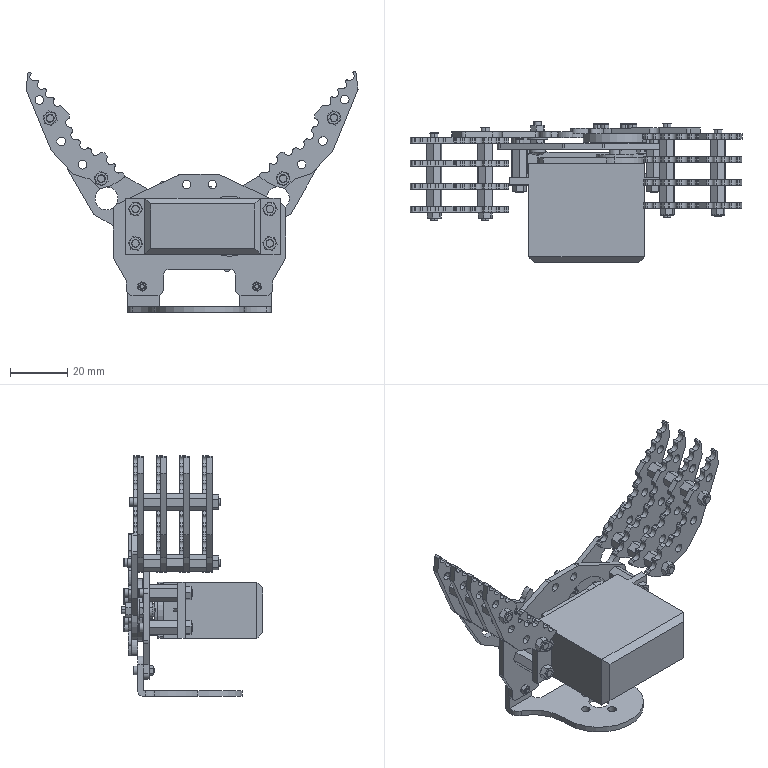Assembly | SolidWorks | mm | 58 component files | 58 solids | 1771 faces | box 115.57 x 49.17 x 83.81 mm | volume 47063 mm3 | plane 747 | cylinder 640 | cone 148 | spline 108 | torus 92 | sphere 36 | commonest cylinder face diameters 3 x232 1 x112 2.5 x110 26.643 x40 4 x34 1.6 x32 22 x16 2 x13
Bill of materials:
3 | 1 |  | Bent flat-plate bracket: rounded, roughly teardrop/bell-shaped base plate with a large central hole and four smaller holes in a square pattern around it, plus two tabs bent up 90 degrees, each with one hole.
4 | 1 |  | Flat plate with an irregular polygonal outline (angled upper edges, two legs below with a rounded rectangular notch between them), one large circular cutout offset to one side, and about ten smaller round holes.
Bolt | 12 |  | Hexagonal prism body with a smaller coaxial cylindrical pin sticking out of one end face, similar in form to a hex standoff with a male end.
cross recessed small pan head screws gb1 | 1 |  | Screw-like part: domed pan-style head with a cross-shaped recess, a short larger-diameter collar under the head, and a long plain cylindrical shank.
hex nuts, style 1-grades ab gb1 | 9 |  | Hexagonal nut form: hex prism with a central round through-bore and chamfered corners on both faces.
hex nuts, style 1-grades ab gb1 | 1 |  | Low-profile hexagonal prism with a central through-bore and a conical chamfer on the corners of one face only. The shape matches a thin hex nut.
hexagon socket head cap screws gb3 | 14 |  | Cap-screw-like part: cylindrical head with a slightly rounded top edge, a shallow circular recess or feature on top, and a long plain cylindrical shank with a chamfered tip.
miniature radial ball bearings gb1 | 1 |  | Flanged ring assembly resembling a flanged ball bearing: outer ring with an external flange on one side, an inner ring, and a single row of balls visible between the rings.
MotorHousing | 1 | CA | Rectangular box-shaped body with chamfered bottom edges, two mounting flanges on opposite ends with two holes each, and a cylindrical boss plus a small raised step on the top face, offset toward one end. The overall form resembles a small actuator housing.
New1 | 1 |  | Flat plate shaped like an arm: a tapered tab with an elongated slot, a large hole and a side notch, joined to a round hub carrying about seven petal-shaped lobes, a central hole and four small holes in a circular pattern.
New1Left | 1 |  | Flat arm-shaped plate: tapered tab with an elongated slot, a large hole and an edge notch, joined to a round hub with about seven petal-shaped lobes, a central hole and four small holes in a circular pattern.
Nut1 | 2 |  | Hexagonal nut form: hex prism with a central round through-bore and chamfered corners on both faces.
PartNew2 | 8 |  | Curved, roughly crescent-shaped flat strip with a row of evenly spaced semicircular scallops along the outer curved edge, a row of five round holes along its length, and a rounded end.
Screw | 4 |  | Hexagonal prism body with a smaller, plain cylindrical stud coming out of one end on the same axis.
Sheet | 1 |  | Flat circular disc flange with four through-holes evenly spaced on a circle, and a solid cylindrical boss or shaft coming out of the center of one face.
Mates:
1. concentric | MotorHousing-1 face at (-24.045, 1.631, 60) dir (0, 1, 0) r 2 | 4-2 face at (-24.045, 8.631, 60) dir (0, 1, 0) r 1.5
2. concentric | MotorHousing-1 face at (22.735, 1.631, 48) dir (0, 1, 0) r 2 | 4-2 face at (22.735, 8.631, 48) dir (0, 1, 0) r 1.5
3. concentric | MotorHousing-1 face at (-24.045, 1.631, 48) dir (0, 1, 0) r 2 | 4-2 face at (-24.045, 8.631, 48) dir (0, 1, 0) r 1.5
4. concentric | MotorHousing-1 face at (-24.045, 1.631, 48) dir (0, 1, 0) r 2 | Screw-2 face at (-24.045, 1.631, 48) dir (0, 1, 0) r 1.25
5. coincident | MotorHousing-1 face at (-0.6553, 6.631, 54) dir (0, 1, 0) | Screw-2 face at (-24.045, 6.631, 48) dir (0, -1, 0)
6. concentric | MotorHousing-1 face at (-24.045, 1.631, 60) dir (0, 1, 0) r 2 | Screw-3 face at (-24.045, 1.631, 60) dir (0, 1, 0) r 1.25
7. coincident | MotorHousing-1 face at (-0.6553, 6.631, 54) dir (0, 1, 0) | Screw-3 face at (-24.045, 6.631, 60) dir (0, -1, 0)
8. concentric | MotorHousing-1 face at (22.735, 1.631, 60) dir (0, 1, 0) r 2 | Screw-4 face at (22.735, 1.631, 60) dir (0, 1, 0) r 1.25
9. concentric | MotorHousing-1 face at (22.735, 1.631, 48) dir (0, 1, 0) r 2 | Screw-5 face at (22.735, 1.631, 48) dir (0, 1, 0) r 1.25
10. coincident | MotorHousing-1 face at (-0.6553, 6.631, 54) dir (0, 1, 0) | Screw-4 face at (22.735, 6.631, 60) dir (0, -1, 0)
11. coincident | MotorHousing-1 face at (-0.6553, 6.631, 54) dir (0, 1, 0) | Screw-5 face at (22.735, 6.631, 48) dir (0, -1, 0)
12. concentric | Screw-2 face at (-24.045, 1.631, 48) dir (0, 1, 0) r 1.25 | hex nuts, style 1-grades ab gb1-1 face at (-24.045, 1.798, 48) dir (0, 1, 0) r 1.25
13. coincident | MotorHousing-1 face at (-0.6553, 4.131, 54) dir (0, -1, 0) | hex nuts, style 1-grades ab gb1-1 face at (-23.062, 4.131, 45.63) dir (0, 1, 0)
14. concentric | Screw-3 face at (-24.045, 1.631, 60) dir (0, 1, 0) r 1.25 | hex nuts, style 1-grades ab gb1-2 face at (-24.045, 1.798, 60) dir (0, 1, 0) r 1.25
15. coincident | MotorHousing-1 face at (-0.6553, 4.131, 54) dir (0, -1, 0) | hex nuts, style 1-grades ab gb1-2 face at (-23.062, 4.131, 57.63) dir (0, 1, 0)
16. coincident | 4-2 face at (-1.765, 16.631, 51) dir (0, -1, 0) | Screw-2 face at (-24.045, 16.631, 48) dir (0, 1, 0)
17. concentric | Screw-4 face at (22.735, 1.631, 60) dir (0, 1, 0) r 1.25 | hex nuts, style 1-grades ab gb1-4 face at (22.735, 1.798, 60) dir (0, 1, 0) r 1.25
18. coincident | Screw-5 face at (22.735, 1.631, 48) dir (0, 1, 0) r 1.25 | hex nuts, style 1-grades ab gb1-3 edge at (22.735, 4.051, 48) dir (0, 1, 0) r 1.25
19. coincident | MotorHousing-1 face at (-0.6553, 4.131, 54) dir (0, -1, 0) | hex nuts, style 1-grades ab gb1-4 edge at (22.735, 4.131, 60) dir (0, -1, 0) r 2.118
20. coincident | MotorHousing-1 face at (-0.6553, 4.131, 54) dir (0, -1, 0) | hex nuts, style 1-grades ab gb1-3 face at (23.718, 4.131, 45.63) dir (0, 1, 0)
21. concentric | 4-2 face at (-24.045, 8.631, 48) dir (0, 1, 0) r 1.5 | hexagon socket head cap screws gb3-2 face at (-24.045, 12.631, 48) dir (0, 1, 0) r 0.8
22. coincident | 4-2 face at (-1.765, 18.631, 51) dir (0, 1, 0) | hexagon socket head cap screws gb3-2 face at (-24.045, 18.631, 48) dir (0, -1, 0)
23. concentric | 4-2 face at (-24.045, 8.631, 60) dir (0, 1, 0) r 1.5 | hexagon socket head cap screws gb3-3 face at (-24.045, 12.631, 60) dir (0, 1, 0) r 0.8
24. coincident | 4-2 face at (-1.765, 18.631, 51) dir (0, 1, 0) | hexagon socket head cap screws gb3-3 face at (-24.045, 18.631, 60) dir (0, -1, 0)
25. concentric | 4-2 face at (22.735, 8.631, 60) dir (0, 1, 0) r 1.5 | hexagon socket head cap screws gb3-4 face at (22.735, 12.631, 60) dir (0, 1, 0) r 0.8
26. coincident | 4-2 face at (-1.765, 18.631, 51) dir (0, 1, 0) | hexagon socket head cap screws gb3-4 face at (22.735, 18.631, 60) dir (0, -1, 0)
27. concentric | 4-2 face at (22.735, 8.631, 48) dir (0, 1, 0) r 1.5 | hexagon socket head cap screws gb3-5 face at (22.735, 12.631, 48) dir (0, 1, 0) r 0.8
28. coincident | 4-2 face at (-1.765, 18.631, 51) dir (0, 1, 0) | hexagon socket head cap screws gb3-5 face at (22.735, 18.631, 48) dir (0, -1, 0)
29. concentric | 4-2 face at (-17.765, 8.631, 54) dir (0, 1, 0) r 2 | cross recessed small pan head screws gb1-1 face at (-17.765, 15.802, 54) dir (0, 1, 0) r 1.389
30. coincident | 4-2 face at (-1.765, 16.631, 51) dir (0, -1, 0) | cross recessed small pan head screws gb1-1 face at (-17.311, 16.631, 55.488) dir (0, 1, 0)
31. concentric | cross recessed small pan head screws gb1-1 face at (-17.765, 15.802, 54) dir (0, 1, 0) r 1.389 | miniature radial ball bearings gb1-1 face at (-17.765, 22.287, 54) dir (0, 1, 0) r 1.5
32. concentric | miniature radial ball bearings gb1-1 face at (-17.765, 22.524, 54) dir (0, 1, 0) r 3 | New1-1 face at (-17.765, 22.649, 54) dir (0, -1, 0) r 3.5
33. coincident | miniature radial ball bearings gb1-1 face at (-14.254, 20.649, 54.795) dir (0, 1, 0) | New1-1 face at (-43.708, 20.649, 80.889) dir (0, -1, 0)
34. concentric | MotorHousing-1 face at (9.195, 9.631, 54) dir (0, 1, 0) r 2.9 | Sheet-1 face at (9.195, 11.961, 54) dir (0, 1, 0) r 2
35. concentric | Sheet-1 face at (3.176, 10.861, 50.426) dir (0, 1, 0) r 1.25 | New1Left-1 face at (3.176, 31.961, 50.426) dir (0, -1, 0) r 1.25
36. concentric | Sheet-1 face at (5.621, 10.861, 60.019) dir (0, 1, 0) r 1.25 | New1Left-1 face at (5.621, 31.961, 60.019) dir (0, -1, 0) r 1.25
37. concentric | Sheet-1 face at (12.769, 10.861, 47.981) dir (0, 1, 0) r 1.25 | New1Left-1 face at (12.769, 31.961, 47.981) dir (0, -1, 0) r 1.25
38. concentric | Sheet-1 face at (15.214, 10.861, 57.574) dir (0, 1, 0) r 1.25 | New1Left-1 face at (15.214, 31.961, 57.574) dir (0, -1, 0) r 1.25
39. coincident | Sheet-1 face at (9.195, 21.961, 54) dir (0, 1, 0) | New1Left-1 face at (35.044, 21.961, 80.978) dir (0, -1, 0)
40. concentric | New1Left-1 face at (3.176, 31.961, 50.426) dir (0, -1, 0) r 1.25 | hexagon socket head cap screws gb3-6 face at (3.176, 17.961, 50.426) dir (0, 1, 0) r 0.8
41. coincident | New1Left-1 face at (35.044, 23.961, 80.978) dir (0, 1, 0) | hexagon socket head cap screws gb3-6 face at (3.176, 23.961, 50.426) dir (0, -1, 0)
42. concentric | New1Left-1 face at (12.769, 31.961, 47.981) dir (0, -1, 0) r 1.25 | hexagon socket head cap screws gb3-7 face at (12.769, 17.961, 47.981) dir (0, 1, 0) r 0.8
43. coincident | New1Left-1 face at (35.044, 23.961, 80.978) dir (0, 1, 0) | hexagon socket head cap screws gb3-7 face at (12.769, 23.961, 47.981) dir (0, -1, 0)
44. concentric | New1Left-1 face at (15.214, 31.961, 57.574) dir (0, -1, 0) r 1.25 | hexagon socket head cap screws gb3-8 face at (15.214, 17.961, 57.574) dir (0, 1, 0) r 0.8
45. coincident | New1Left-1 face at (35.044, 23.961, 80.978) dir (0, 1, 0) | hexagon socket head cap screws gb3-8 face at (15.214, 23.961, 57.574) dir (0, -1, 0)
46. concentric | New1Left-1 face at (5.621, 31.961, 60.019) dir (0, -1, 0) r 1.25 | hexagon socket head cap screws gb3-9 face at (5.621, 17.961, 60.019) dir (0, 1, 0) r 0.8
47. coincident | New1Left-1 face at (35.044, 23.961, 80.978) dir (0, 1, 0) | hexagon socket head cap screws gb3-9 face at (5.621, 23.961, 60.019) dir (0, -1, 0)
48. distance | MotorHousing-1 face at (9.195, 9.631, 54) dir (0, 1, 0) | Sheet-1 face at (9.195, 11.961, 54) dir (0, -1, 0)
49. concentric | PartNew2-1 face at (-35.954, -3.351, 70.518) dir (0, -1, 0) r 1.5 | Bolt-1 face at (-35.954, -8.351, 70.518) dir (0, 1, 0) r 1.25
50. coincident | PartNew2-1 face at (39.001, -3.351, 96.421) dir (0, 1, 0) | Bolt-1 face at (-35.954, -3.351, 70.518) dir (0, -1, 0)
51. concentric | PartNew2-1 face at (-53.757, -3.351, 91.594) dir (0, -1, 0) r 1.5 | Bolt-2 face at (-53.757, -8.351, 91.594) dir (0, 1, 0) r 1.25
52. coincident | PartNew2-1 face at (39.001, -3.351, 96.421) dir (0, 1, 0) | Bolt-2 face at (-53.757, -3.351, 91.594) dir (0, -1, 0)
53. concentric | Bolt-1 face at (-35.954, -2.351, 70.518) dir (0, 1, 0) r 1.25 | PartNew2-2 face at (-35.954, 4.649, 70.518) dir (0, -1, 0) r 1.5
54. concentric | Bolt-2 face at (-53.757, -2.351, 91.594) dir (0, 1, 0) r 1.25 | PartNew2-2 face at (-53.757, 4.649, 91.594) dir (0, -1, 0) r 1.5
55. coincident | Bolt-1 face at (-35.954, 2.649, 70.518) dir (0, 1, 0) | PartNew2-2 face at (39.001, 2.649, 96.421) dir (0, -1, 0)
56. concentric | PartNew2-2 face at (-35.954, 4.649, 70.518) dir (0, -1, 0) r 1.5 | Bolt-3 face at (-35.954, -0.3506, 70.518) dir (0, 1, 0) r 1.25
57. coincident | PartNew2-2 face at (39.001, 4.649, 96.421) dir (0, 1, 0) | Bolt-3 face at (-35.954, 4.649, 70.518) dir (0, -1, 0)
58. concentric | PartNew2-2 face at (-53.757, 4.649, 91.594) dir (0, -1, 0) r 1.5 | Bolt-4 face at (-53.757, -0.3506, 91.594) dir (0, 1, 0) r 1.25
59. coincident | PartNew2-2 face at (39.001, 4.649, 96.421) dir (0, 1, 0) | Bolt-4 face at (-53.757, 4.649, 91.594) dir (0, -1, 0)
60. concentric | Bolt-3 face at (-35.954, 5.649, 70.518) dir (0, 1, 0) r 1.25 | PartNew2-3 face at (-35.954, 12.649, 70.518) dir (0, -1, 0) r 1.5
61. concentric | Bolt-4 face at (-53.757, 5.649, 91.594) dir (0, 1, 0) r 1.25 | PartNew2-3 face at (-53.757, 12.649, 91.594) dir (0, -1, 0) r 1.5
62. coincident | Bolt-3 face at (-35.954, 10.649, 70.518) dir (0, 1, 0) | PartNew2-3 face at (39.001, 10.649, 96.421) dir (0, -1, 0)
63. concentric | PartNew2-3 face at (-35.954, 12.649, 70.518) dir (0, -1, 0) r 1.5 | Bolt-5 face at (-35.954, 7.649, 70.518) dir (0, 1, 0) r 1.25
64. concentric | PartNew2-3 face at (-53.757, 12.649, 91.594) dir (0, -1, 0) r 1.5 | Bolt-6 face at (-53.757, 7.649, 91.594) dir (0, 1, 0) r 1.25
65. coincident | PartNew2-3 face at (39.001, 12.649, 96.421) dir (0, 1, 0) | Bolt-5 face at (-35.954, 12.649, 70.518) dir (0, -1, 0)
66. coincident | PartNew2-3 face at (39.001, 12.649, 96.421) dir (0, 1, 0) | Bolt-6 face at (-53.757, 12.649, 91.594) dir (0, -1, 0)
67. concentric | Bolt-5 face at (-35.954, 13.649, 70.518) dir (0, 1, 0) r 1.25 | PartNew2-4 face at (-35.954, 20.649, 70.518) dir (0, -1, 0) r 1.5
68. concentric | Bolt-6 face at (-53.757, 13.649, 91.594) dir (0, 1, 0) r 1.25 | PartNew2-4 face at (-53.757, 20.649, 91.594) dir (0, -1, 0) r 1.5
69. coincident | Bolt-5 face at (-35.954, 18.649, 70.518) dir (0, 1, 0) | PartNew2-4 face at (39.001, 18.649, 96.421) dir (0, -1, 0)
70. concentric | New1-1 face at (-35.954, 22.649, 70.518) dir (0, -1, 0) r 1.5 | PartNew2-4 face at (-35.954, 20.649, 70.518) dir (0, -1, 0) r 1.5
71. tangent | New1-1 face at (-46.794, 22.649, 76.776) dir (0.6002, 0, 0.7999) | PartNew2-4 face at (-42.465, 20.649, 75.403) dir (0, -1, 0) r 1.5
72. concentric | PartNew2-5 face at (27.326, -4.039, 70.581) dir (0, 1, 0) r 1.5 | Bolt-7 face at (27.326, -7.039, 70.581) dir (0, 1, 0) r 1.25
73. concentric | PartNew2-5 face at (45.055, -4.039, 91.719) dir (0, 1, 0) r 1.5 | Bolt-8 face at (45.055, -7.039, 91.719) dir (0, 1, 0) r 1.25
74. coincident | PartNew2-5 face at (-47.719, -2.039, 96.224) dir (0, 1, 0) | Bolt-7 face at (27.326, -2.039, 70.581) dir (0, -1, 0)
75. coincident | PartNew2-5 face at (-47.719, -2.039, 96.224) dir (0, 1, 0) | Bolt-8 face at (45.055, -2.039, 91.719) dir (0, -1, 0)
76. concentric | Bolt-7 face at (27.326, -1.039, 70.581) dir (0, 1, 0) r 1.25 | PartNew2-6 face at (27.326, 3.961, 70.581) dir (0, 1, 0) r 1.5
77. concentric | Bolt-8 face at (45.055, -1.039, 91.719) dir (0, 1, 0) r 1.25 | PartNew2-6 face at (45.055, 3.961, 91.719) dir (0, 1, 0) r 1.5
78. coincident | Bolt-7 face at (27.326, 3.961, 70.581) dir (0, 1, 0) | PartNew2-6 face at (-47.719, 3.961, 96.224) dir (0, -1, 0)
79. concentric | PartNew2-6 face at (27.326, 3.961, 70.581) dir (0, 1, 0) r 1.5 | Bolt-9 face at (27.326, 0.961, 70.581) dir (0, 1, 0) r 1.25
80. concentric | PartNew2-6 face at (45.055, 3.961, 91.719) dir (0, 1, 0) r 1.5 | Bolt-10 face at (45.055, 0.961, 91.719) dir (0, 1, 0) r 1.25
81. coincident | PartNew2-6 face at (-47.719, 5.961, 96.224) dir (0, 1, 0) | Bolt-9 face at (27.326, 5.961, 70.581) dir (0, -1, 0)
82. coincident | PartNew2-6 face at (-47.719, 5.961, 96.224) dir (0, 1, 0) | Bolt-10 face at (45.055, 5.961, 91.719) dir (0, -1, 0)
83. concentric | Bolt-9 face at (27.326, 6.961, 70.581) dir (0, 1, 0) r 1.25 | PartNew2-7 face at (27.326, 11.961, 70.581) dir (0, 1, 0) r 1.5
84. concentric | Bolt-10 face at (45.055, 6.961, 91.719) dir (0, 1, 0) r 1.25 | PartNew2-7 face at (45.055, 11.961, 91.719) dir (0, 1, 0) r 1.5
85. coincident | Bolt-9 face at (27.326, 11.961, 70.581) dir (0, 1, 0) | PartNew2-7 face at (-47.719, 11.961, 96.224) dir (0, -1, 0)
86. concentric | PartNew2-7 face at (27.326, 11.961, 70.581) dir (0, 1, 0) r 1.5 | Bolt-11 face at (27.326, 8.961, 70.581) dir (0, 1, 0) r 1.25
87. concentric | PartNew2-7 face at (45.055, 11.961, 91.719) dir (0, 1, 0) r 1.5 | Bolt-12 face at (45.055, 8.961, 91.719) dir (0, 1, 0) r 1.25
88. coincident | PartNew2-7 face at (-47.719, 13.961, 96.224) dir (0, 1, 0) | Bolt-11 face at (27.326, 13.961, 70.581) dir (0, -1, 0)
89. coincident | PartNew2-7 face at (-47.719, 13.961, 96.224) dir (0, 1, 0) | Bolt-12 face at (45.055, 13.961, 91.719) dir (0, -1, 0)
90. concentric | Bolt-11 face at (27.326, 14.961, 70.581) dir (0, 1, 0) r 1.25 | PartNew2-8 face at (27.326, 19.961, 70.581) dir (0, 1, 0) r 1.5
91. concentric | Bolt-12 face at (45.055, 14.961, 91.719) dir (0, 1, 0) r 1.25 | PartNew2-8 face at (45.055, 19.961, 91.719) dir (0, 1, 0) r 1.5
92. coincident | Bolt-11 face at (27.326, 19.961, 70.581) dir (0, 1, 0) | PartNew2-8 face at (-47.719, 19.961, 96.224) dir (0, -1, 0)
93. concentric | New1Left-1 face at (27.326, 21.961, 70.581) dir (0, 1, 0) r 1.5 | PartNew2-8 face at (27.326, 19.961, 70.581) dir (0, 1, 0) r 1.5
94. coincident | New1Left-1 face at (35.044, 21.961, 80.978) dir (0, -1, 0) | PartNew2-8 face at (-47.719, 21.961, 96.224) dir (0, 1, 0)
95. tangent | New1Left-1 face at (38.144, 21.961, 76.876) dir (-0.6029, 0, 0.7978) | PartNew2-8 face at (33.82, 19.961, 75.489) dir (0, 1, 0) r 1.5
96. coincident | New1-1 face at (-43.708, 20.649, 80.889) dir (0, -1, 0) | PartNew2-4 face at (39.001, 20.649, 96.421) dir (0, 1, 0)
97. concentric | New1-1 face at (-35.954, 22.649, 70.518) dir (0, -1, 0) r 1.5 | hexagon socket head cap screws gb3-10 face at (-35.954, 16.649, 70.518) dir (0, 1, 0) r 0.8
98. coincident | New1-1 face at (-43.708, 22.649, 80.889) dir (0, 1, 0) | hexagon socket head cap screws gb3-10 face at (-35.954, 22.649, 70.518) dir (0, -1, 0)
99. concentric | PartNew2-4 face at (-53.757, 20.649, 91.594) dir (0, -1, 0) r 1.5 | hexagon socket head cap screws gb3-11 face at (-53.757, 14.649, 91.594) dir (0, 1, 0) r 0.8
100. coincident | PartNew2-4 face at (39.001, 20.649, 96.421) dir (0, 1, 0) | hexagon socket head cap screws gb3-11 face at (-53.757, 20.649, 91.594) dir (0, -1, 0)
101. concentric | New1Left-1 face at (27.326, 21.961, 70.581) dir (0, 1, 0) r 1.5 | hexagon socket head cap screws gb3-12 face at (27.326, 17.961, 70.581) dir (0, 1, 0) r 0.8
102. coincident | New1Left-1 face at (35.044, 23.961, 80.978) dir (0, 1, 0) | hexagon socket head cap screws gb3-12 face at (27.326, 23.961, 70.581) dir (0, -1, 0)
103. concentric | PartNew2-8 face at (45.055, 19.961, 91.719) dir (0, 1, 0) r 1.5 | hexagon socket head cap screws gb3-13 face at (45.055, 15.961, 91.719) dir (0, 1, 0) r 0.8
104. coincident | PartNew2-8 face at (-47.719, 21.961, 96.224) dir (0, 1, 0) | hexagon socket head cap screws gb3-13 face at (45.055, 21.961, 91.719) dir (0, -1, 0)
105. concentric | PartNew2-1 face at (-35.954, -3.351, 70.518) dir (0, -1, 0) r 1.5 | hex nuts, style 1-grades ab gb1-6 face at (-35.954, -5.351, 70.518) dir (0, -1, 0) r 523.599
106. coincident | PartNew2-1 face at (39.001, -5.351, 96.421) dir (0, -1, 0) | hex nuts, style 1-grades ab gb1-6 face at (-36.428, -5.351, 73.04) dir (0, 1, 0)
107. concentric | PartNew2-1 face at (-53.757, -3.351, 91.594) dir (0, -1, 0) r 1.5 | hex nuts, style 1-grades ab gb1-7 face at (-53.757, -5.351, 91.594) dir (0, -1, 0) r 523.599
108. coincident | PartNew2-1 face at (39.001, -5.351, 96.421) dir (0, -1, 0) | hex nuts, style 1-grades ab gb1-7 face at (-54.23, -5.351, 94.116) dir (0, 1, 0)
109. concentric | PartNew2-5 face at (27.326, -4.039, 70.581) dir (0, 1, 0) r 1.5 | hex nuts, style 1-grades ab gb1-10 face at (27.326, -4.039, 70.581) dir (0, -1, 0) r 523.599
110. coincident | PartNew2-5 face at (-47.719, -4.039, 96.224) dir (0, -1, 0) | hex nuts, style 1-grades ab gb1-10 face at (26.853, -4.039, 73.103) dir (0, 1, 0)
111. concentric | PartNew2-5 face at (45.055, -4.039, 91.719) dir (0, 1, 0) r 1.5 | hex nuts, style 1-grades ab gb1-11 face at (45.055, -4.039, 91.719) dir (0, -1, 0) r 523.599
112. coincident | PartNew2-5 face at (-47.719, -4.039, 96.224) dir (0, -1, 0) | hex nuts, style 1-grades ab gb1-11 face at (44.582, -4.039, 94.241) dir (0, 1, 0)
113. concentric | 4-2 face at (18.235, 8.631, 33) dir (0, 1, 0) r 1.5 | 3-1 face at (18.235, -0.369, 33) dir (0, 1, 0) r 1.5
114. concentric | 4-2 face at (-21.765, 8.631, 33) dir (0, 1, 0) r 1.5 | 3-1 face at (-21.765, -0.369, 33) dir (0, 1, 0) r 1.5
115. coincident | 4-2 face at (-1.765, 18.631, 51) dir (0, 1, 0) | 3-1 face at (-15.765, 18.631, 38) dir (0, -1, 0)
116. concentric | 3-1 face at (18.235, -0.369, 33) dir (0, 1, 0) r 1.5 | hexagon socket head cap screws gb3-14 face at (18.235, 14.631, 33) dir (0, 1, 0) r 0.8
117. coincident | 3-1 face at (12.235, 20.631, 26) dir (0, 1, 0) | hexagon socket head cap screws gb3-14 face at (18.235, 20.631, 33) dir (0, -1, 0)
118. concentric | 3-1 face at (-21.765, -0.369, 33) dir (0, 1, 0) r 1.5 | hexagon socket head cap screws gb3-15 face at (-21.765, 14.631, 33) dir (0, 1, 0) r 0.8
119. coincident | 3-1 face at (-26.765, 20.631, 26) dir (0, 1, 0) | hexagon socket head cap screws gb3-15 face at (-21.765, 20.631, 33) dir (0, -1, 0)
120. coincident | 4-2 face at (-1.765, 18.631, 51) dir (0, 1, 0) | hex nuts, style 1-grades ab gb1-12 face at (-18.239, 18.631, 56.522) dir (0, -1, 0)
121. concentric | cross recessed small pan head screws gb1-1 face at (-17.765, 15.802, 54) dir (0, 1, 0) r 1.389 | hex nuts, style 1-grades ab gb1-13 face at (-17.765, 24.983, 54) dir (0, -1, 0) r 1.25
122. coincident | New1-1 face at (-43.708, 22.649, 80.889) dir (0, 1, 0) | hex nuts, style 1-grades ab gb1-13 face at (-18.239, 22.649, 56.522) dir (0, -1, 0)
123. concentric | hexagon socket head cap screws gb3-15 face at (-21.765, 14.631, 33) dir (0, 1, 0) r 0.8 | Nut1-5 face at (-21.765, 16.631, 33) dir (0, -1, 0) r 0.8
124. coincident | 4-2 face at (-1.765, 16.631, 51) dir (0, -1, 0) | Nut1-5 edge at (-21.765, 16.631, 33) dir (0, 1, 0) r 1.356
125. concentric | hexagon socket head cap screws gb3-14 face at (18.235, 14.631, 33) dir (0, 1, 0) r 0.8 | Nut1-6 face at (18.235, 16.631, 33) dir (0, -1, 0) r 0.8
126. coincident | 4-2 face at (-1.765, 16.631, 51) dir (0, -1, 0) | Nut1-6 face at (19.752, 16.631, 32.371) dir (0, 1, 0)
127. concentric | cross recessed small pan head screws gb1-1 face at (-17.765, 15.802, 54) dir (0, 1, 0) r 1.389 | hex nuts, style 1-grades ab gb1-12 face at (-17.765, 20.964, 54) dir (0, -1, 0) r 1.25